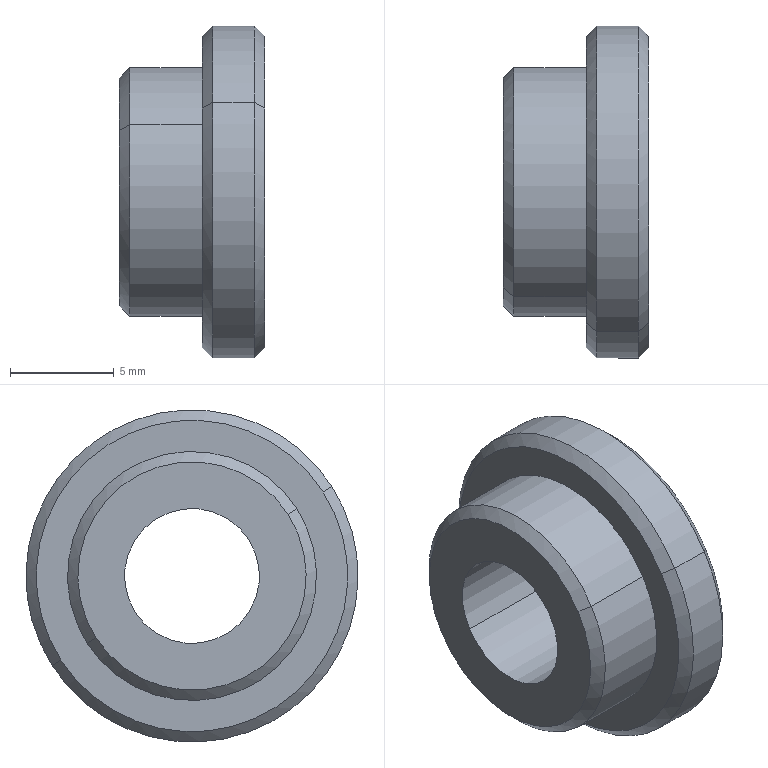Component | SolidWorks | RetainingRing-1 | 1 solid | 15 faces | box 7 x 16 x 16 mm | volume 806 mm3 | cone 6 | cylinder 6 | plane 3 | commonest cylinder face diameters 12 x2 16 x2 6.5 x2
build123d program:
from build123d import *


with BuildPart() as part:
    # Sketch1 → Revolve1 (revolve)
    with BuildSketch(Plane(origin=(0, 0, 0), x_dir=(0, 0, -1), z_dir=(1, 0, 0)), mode=Mode.PRIVATE) as revolve1_sk:
        Polygon((0, 3.25), (0, 7.5), (0.5, 8), (2.5, 8), (3, 7.5), (3, 6), (6.5, 6), (7, 5.5), (7, 3.25), align=None)
    revolve(revolve1_sk.sketch.rotate(Axis((0, 0, 0), (0, 0, -1)), 90), axis=Axis((0, 0, 0), (0, 0, -1)))


solid = part.part

# Placed as in the assembly
solid = solid.moved(Location((120.296, 56.837, 344.838), (0, 90, 0)))
STEP:
#1=COLOUR_RGB('',0.7922,0.8196,0.9333);
#2=FILL_AREA_STYLE_COLOUR('',#1);
#3=FILL_AREA_STYLE('',(#2));
#4=SURFACE_STYLE_FILL_AREA(#3);
#5=SURFACE_SIDE_STYLE('',(#4));
#6=SURFACE_STYLE_USAGE(.BOTH.,#5);
#7=PRESENTATION_STYLE_ASSIGNMENT((#6));
#8=CARTESIAN_POINT('',(4.46,2.055,13.693));
#9=VERTEX_POINT('',#8);
#10=CARTESIAN_POINT('',(4.46,2.42,13.459));
#11=VERTEX_POINT('',#10);
#12=CARTESIAN_POINT('',(4.46,2.238,13.576));
#13=DIRECTION('',(1.,0.,-0.));
#14=DIRECTION('',(0.,-0.8419,0.5397));
#15=AXIS2_PLACEMENT_3D('',#12,#13,#14);
#16=CIRCLE('',#15,0.2165);
#17=EDGE_CURVE('',#9,#11,#16,.T.);
#18=ORIENTED_EDGE('',*,*,#17,.T.);
#19=CARTESIAN_POINT('',(4.48,2.437,13.449));
#20=VERTEX_POINT('',#19);
#21=CARTESIAN_POINT('',(4.46,2.42,13.459));
#22=DIRECTION('',(0.7071,0.5953,-0.3816));
#23=VECTOR('',#22,39.37);
#24=LINE('',#21,#23);
#25=EDGE_CURVE('',#11,#20,#24,.T.);
#26=ORIENTED_EDGE('',*,*,#25,.T.);
#27=CARTESIAN_POINT('',(4.48,2.039,13.704));
#28=VERTEX_POINT('',#27);
#29=CARTESIAN_POINT('',(4.48,2.238,13.576));
#30=DIRECTION('',(1.,0.,-0.));
#31=DIRECTION('',(0.,-0.8419,0.5397));
#32=AXIS2_PLACEMENT_3D('',#29,#30,#31);
#33=CIRCLE('',#32,0.2362);
#34=EDGE_CURVE('',#28,#20,#33,.T.);
#35=ORIENTED_EDGE('',*,*,#34,.F.);
#36=CARTESIAN_POINT('',(4.46,2.055,13.693));
#37=DIRECTION('',(0.7071,-0.5953,0.3816));
#38=VECTOR('',#37,39.37);
#39=LINE('',#36,#38);
#40=EDGE_CURVE('',#9,#28,#39,.T.);
#41=ORIENTED_EDGE('',*,*,#40,.F.);
#42=EDGE_LOOP('',(#18,#26,#35,#41));
#43=FACE_OUTER_BOUND('',#42,.T.);
#44=CARTESIAN_POINT('',(4.46,2.238,13.576));
#45=DIRECTION('',(1.,0.,-0.));
#46=DIRECTION('',(0.,-0.8419,0.5397));
#47=AXIS2_PLACEMENT_3D('',#44,#45,#46);
#48=CONICAL_SURFACE('',#47,0.2165,0.7854);
#49=ADVANCED_FACE('',(#43),#48,.T.);
#50=ORIENTED_EDGE('',*,*,#34,.T.);
#51=CARTESIAN_POINT('',(4.618,2.437,13.449));
#52=VERTEX_POINT('',#51);
#53=CARTESIAN_POINT('',(4.736,2.437,13.449));
#54=DIRECTION('',(1.,0.,-0.));
#55=VECTOR('',#54,39.37);
#56=LINE('',#53,#55);
#57=EDGE_CURVE('',#20,#52,#56,.T.);
#58=ORIENTED_EDGE('',*,*,#57,.T.);
#59=CARTESIAN_POINT('',(4.618,2.039,13.704));
#60=VERTEX_POINT('',#59);
#61=CARTESIAN_POINT('',(4.618,2.238,13.576));
#62=DIRECTION('',(1.,0.,-0.));
#63=DIRECTION('',(0.,-0.8419,0.5397));
#64=AXIS2_PLACEMENT_3D('',#61,#62,#63);
#65=CIRCLE('',#64,0.2362);
#66=EDGE_CURVE('',#60,#52,#65,.T.);
#67=ORIENTED_EDGE('',*,*,#66,.F.);
#68=CARTESIAN_POINT('',(4.736,2.039,13.704));
#69=DIRECTION('',(1.,0.,-0.));
#70=VECTOR('',#69,39.37);
#71=LINE('',#68,#70);
#72=EDGE_CURVE('',#28,#60,#71,.T.);
#73=ORIENTED_EDGE('',*,*,#72,.F.);
#74=EDGE_LOOP('',(#50,#58,#67,#73));
#75=FACE_OUTER_BOUND('',#74,.T.);
#76=CARTESIAN_POINT('',(4.736,2.238,13.576));
#77=DIRECTION('',(1.,0.,-0.));
#78=DIRECTION('',(0.,-0.8419,0.5397));
#79=AXIS2_PLACEMENT_3D('',#76,#77,#78);
#80=CYLINDRICAL_SURFACE('',#79,0.2362);
#81=ADVANCED_FACE('',(#75),#80,.T.);
#82=CARTESIAN_POINT('',(4.618,1.989,13.736));
#83=VERTEX_POINT('',#82);
#84=CARTESIAN_POINT('',(4.618,2.486,13.417));
#85=VERTEX_POINT('',#84);
#86=CARTESIAN_POINT('',(4.618,2.238,13.576));
#87=DIRECTION('',(1.,0.,-0.));
#88=DIRECTION('',(0.,-0.8419,0.5397));
#89=AXIS2_PLACEMENT_3D('',#86,#87,#88);
#90=CIRCLE('',#89,0.2953);
#91=EDGE_CURVE('',#83,#85,#90,.T.);
#92=ORIENTED_EDGE('',*,*,#91,.T.);
#93=CARTESIAN_POINT('',(4.638,2.503,13.406));
#94=VERTEX_POINT('',#93);
#95=CARTESIAN_POINT('',(4.618,2.486,13.417));
#96=DIRECTION('',(0.7071,0.5953,-0.3816));
#97=VECTOR('',#96,39.37);
#98=LINE('',#95,#97);
#99=EDGE_CURVE('',#85,#94,#98,.T.);
#100=ORIENTED_EDGE('',*,*,#99,.T.);
#101=CARTESIAN_POINT('',(4.638,1.973,13.746));
#102=VERTEX_POINT('',#101);
#103=CARTESIAN_POINT('',(4.638,2.238,13.576));
#104=DIRECTION('',(1.,0.,-0.));
#105=DIRECTION('',(0.,-0.8419,0.5397));
#106=AXIS2_PLACEMENT_3D('',#103,#104,#105);
#107=CIRCLE('',#106,0.315);
#108=EDGE_CURVE('',#102,#94,#107,.T.);
#109=ORIENTED_EDGE('',*,*,#108,.F.);
#110=CARTESIAN_POINT('',(4.618,1.989,13.736));
#111=DIRECTION('',(0.7071,-0.5953,0.3816));
#112=VECTOR('',#111,39.37);
#113=LINE('',#110,#112);
#114=EDGE_CURVE('',#83,#102,#113,.T.);
#115=ORIENTED_EDGE('',*,*,#114,.F.);
#116=EDGE_LOOP('',(#92,#100,#109,#115));
#117=FACE_OUTER_BOUND('',#116,.T.);
#118=CARTESIAN_POINT('',(4.618,2.238,13.576));
#119=DIRECTION('',(1.,0.,-0.));
#120=DIRECTION('',(0.,-0.8419,0.5397));
#121=AXIS2_PLACEMENT_3D('',#118,#119,#120);
#122=CONICAL_SURFACE('',#121,0.2953,0.7854);
#123=ADVANCED_FACE('',(#117),#122,.T.);
#124=ORIENTED_EDGE('',*,*,#108,.T.);
#125=CARTESIAN_POINT('',(4.716,2.503,13.406));
#126=VERTEX_POINT('',#125);
#127=CARTESIAN_POINT('',(4.736,2.503,13.406));
#128=DIRECTION('',(1.,0.,-0.));
#129=VECTOR('',#128,39.37);
#130=LINE('',#127,#129);
#131=EDGE_CURVE('',#94,#126,#130,.T.);
#132=ORIENTED_EDGE('',*,*,#131,.T.);
#133=CARTESIAN_POINT('',(4.716,1.973,13.746));
#134=VERTEX_POINT('',#133);
#135=CARTESIAN_POINT('',(4.716,2.238,13.576));
#136=DIRECTION('',(1.,0.,-0.));
#137=DIRECTION('',(0.,-0.8419,0.5397));
#138=AXIS2_PLACEMENT_3D('',#135,#136,#137);
#139=CIRCLE('',#138,0.315);
#140=EDGE_CURVE('',#134,#126,#139,.T.);
#141=ORIENTED_EDGE('',*,*,#140,.F.);
#142=CARTESIAN_POINT('',(4.736,1.973,13.746));
#143=DIRECTION('',(1.,0.,-0.));
#144=VECTOR('',#143,39.37);
#145=LINE('',#142,#144);
#146=EDGE_CURVE('',#102,#134,#145,.T.);
#147=ORIENTED_EDGE('',*,*,#146,.F.);
#148=EDGE_LOOP('',(#124,#132,#141,#147));
#149=FACE_OUTER_BOUND('',#148,.T.);
#150=CARTESIAN_POINT('',(4.736,2.238,13.576));
#151=DIRECTION('',(1.,0.,-0.));
#152=DIRECTION('',(0.,-0.8419,0.5397));
#153=AXIS2_PLACEMENT_3D('',#150,#151,#152);
#154=CYLINDRICAL_SURFACE('',#153,0.315);
#155=ADVANCED_FACE('',(#149),#154,.T.);
#156=CARTESIAN_POINT('',(4.736,1.989,13.736));
#157=VERTEX_POINT('',#156);
#158=CARTESIAN_POINT('',(4.736,2.486,13.417));
#159=VERTEX_POINT('',#158);
#160=CARTESIAN_POINT('',(4.736,2.238,13.576));
#161=DIRECTION('',(1.,0.,-0.));
#162=DIRECTION('',(0.,-0.8419,0.5397));
#163=AXIS2_PLACEMENT_3D('',#160,#161,#162);
#164=CIRCLE('',#163,0.2953);
#165=EDGE_CURVE('',#157,#159,#164,.T.);
#166=ORIENTED_EDGE('',*,*,#165,.F.);
#167=CARTESIAN_POINT('',(4.716,1.973,13.746));
#168=DIRECTION('',(-0.7071,-0.5953,0.3816));
#169=VECTOR('',#168,39.37);
#170=LINE('',#167,#169);
#171=EDGE_CURVE('',#157,#134,#170,.T.);
#172=ORIENTED_EDGE('',*,*,#171,.T.);
#173=ORIENTED_EDGE('',*,*,#140,.T.);
#174=CARTESIAN_POINT('',(4.716,2.503,13.406));
#175=DIRECTION('',(-0.7071,0.5953,-0.3816));
#176=VECTOR('',#175,39.37);
#177=LINE('',#174,#176);
#178=EDGE_CURVE('',#159,#126,#177,.T.);
#179=ORIENTED_EDGE('',*,*,#178,.F.);
#180=EDGE_LOOP('',(#166,#172,#173,#179));
#181=FACE_OUTER_BOUND('',#180,.T.);
#182=CARTESIAN_POINT('',(4.716,2.238,13.576));
#183=DIRECTION('',(-1.,-0.,0.));
#184=DIRECTION('',(-0.,0.8419,-0.5397));
#185=AXIS2_PLACEMENT_3D('',#182,#183,#184);
#186=CONICAL_SURFACE('',#185,0.315,0.7854);
#187=ADVANCED_FACE('',(#181),#186,.T.);
#188=CARTESIAN_POINT('',(4.46,2.345,13.507));
#189=VERTEX_POINT('',#188);
#190=CARTESIAN_POINT('',(4.46,2.13,13.645));
#191=VERTEX_POINT('',#190);
#192=CARTESIAN_POINT('',(4.46,2.238,13.576));
#193=DIRECTION('',(1.,0.,-0.));
#194=DIRECTION('',(0.,-0.8419,0.5397));
#195=AXIS2_PLACEMENT_3D('',#192,#193,#194);
#196=CIRCLE('',#195,0.128);
#197=EDGE_CURVE('',#189,#191,#196,.T.);
#198=ORIENTED_EDGE('',*,*,#197,.F.);
#199=CARTESIAN_POINT('',(4.736,2.345,13.507));
#200=VERTEX_POINT('',#199);
#201=CARTESIAN_POINT('',(4.736,2.345,13.507));
#202=DIRECTION('',(1.,0.,-0.));
#203=VECTOR('',#202,39.37);
#204=LINE('',#201,#203);
#205=EDGE_CURVE('',#189,#200,#204,.T.);
#206=ORIENTED_EDGE('',*,*,#205,.T.);
#207=CARTESIAN_POINT('',(4.736,2.13,13.645));
#208=VERTEX_POINT('',#207);
#209=CARTESIAN_POINT('',(4.736,2.238,13.576));
#210=DIRECTION('',(1.,0.,-0.));
#211=DIRECTION('',(0.,-0.8419,0.5397));
#212=AXIS2_PLACEMENT_3D('',#209,#210,#211);
#213=CIRCLE('',#212,0.128);
#214=EDGE_CURVE('',#200,#208,#213,.T.);
#215=ORIENTED_EDGE('',*,*,#214,.T.);
#216=CARTESIAN_POINT('',(4.736,2.13,13.645));
#217=DIRECTION('',(1.,0.,-0.));
#218=VECTOR('',#217,39.37);
#219=LINE('',#216,#218);
#220=EDGE_CURVE('',#191,#208,#219,.T.);
#221=ORIENTED_EDGE('',*,*,#220,.F.);
#222=EDGE_LOOP('',(#198,#206,#215,#221));
#223=FACE_OUTER_BOUND('',#222,.T.);
#224=CARTESIAN_POINT('',(4.736,2.238,13.576));
#225=DIRECTION('',(1.,0.,-0.));
#226=DIRECTION('',(0.,-0.8419,0.5397));
#227=AXIS2_PLACEMENT_3D('',#224,#225,#226);
#228=CYLINDRICAL_SURFACE('',#227,0.128);
#229=ADVANCED_FACE('',(#223),#228,.F.);
#230=ORIENTED_EDGE('',*,*,#205,.F.);
#231=CARTESIAN_POINT('',(4.46,2.238,13.576));
#232=DIRECTION('',(1.,0.,-0.));
#233=DIRECTION('',(0.,-0.8419,0.5397));
#234=AXIS2_PLACEMENT_3D('',#231,#232,#233);
#235=CIRCLE('',#234,0.128);
#236=EDGE_CURVE('',#191,#189,#235,.T.);
#237=ORIENTED_EDGE('',*,*,#236,.F.);
#238=ORIENTED_EDGE('',*,*,#220,.T.);
#239=CARTESIAN_POINT('',(4.736,2.238,13.576));
#240=DIRECTION('',(1.,0.,-0.));
#241=DIRECTION('',(0.,-0.8419,0.5397));
#242=AXIS2_PLACEMENT_3D('',#239,#240,#241);
#243=CIRCLE('',#242,0.128);
#244=EDGE_CURVE('',#208,#200,#243,.T.);
#245=ORIENTED_EDGE('',*,*,#244,.T.);
#246=EDGE_LOOP('',(#230,#237,#238,#245));
#247=FACE_OUTER_BOUND('',#246,.T.);
#248=CARTESIAN_POINT('',(4.736,2.238,13.576));
#249=DIRECTION('',(1.,0.,-0.));
#250=DIRECTION('',(0.,-0.8419,0.5397));
#251=AXIS2_PLACEMENT_3D('',#248,#249,#250);
#252=CYLINDRICAL_SURFACE('',#251,0.128);
#253=ADVANCED_FACE('',(#247),#252,.F.);
#254=ORIENTED_EDGE('',*,*,#244,.F.);
#255=ORIENTED_EDGE('',*,*,#214,.F.);
#256=EDGE_LOOP('',(#254,#255));
#257=FACE_BOUND('',#256,.T.);
#258=CARTESIAN_POINT('',(4.736,2.238,13.576));
#259=DIRECTION('',(1.,0.,-0.));
#260=DIRECTION('',(0.,-0.8419,0.5397));
#261=AXIS2_PLACEMENT_3D('',#258,#259,#260);
#262=CIRCLE('',#261,0.2953);
#263=EDGE_CURVE('',#159,#157,#262,.T.);
#264=ORIENTED_EDGE('',*,*,#263,.T.);
#265=ORIENTED_EDGE('',*,*,#165,.T.);
#266=EDGE_LOOP('',(#264,#265));
#267=FACE_OUTER_BOUND('',#266,.T.);
#268=CARTESIAN_POINT('',(4.736,2.169,13.469));
#269=DIRECTION('',(-1.,-0.,0.));
#270=DIRECTION('',(-0.,0.8419,-0.5397));
#271=AXIS2_PLACEMENT_3D('',#268,#269,#270);
#272=PLANE('',#271);
#273=ADVANCED_FACE('',(#257,#267),#272,.F.);
#274=ORIENTED_EDGE('',*,*,#171,.F.);
#275=ORIENTED_EDGE('',*,*,#263,.F.);
#276=ORIENTED_EDGE('',*,*,#178,.T.);
#277=CARTESIAN_POINT('',(4.716,2.238,13.576));
#278=DIRECTION('',(1.,0.,-0.));
#279=DIRECTION('',(0.,-0.8419,0.5397));
#280=AXIS2_PLACEMENT_3D('',#277,#278,#279);
#281=CIRCLE('',#280,0.315);
#282=EDGE_CURVE('',#126,#134,#281,.T.);
#283=ORIENTED_EDGE('',*,*,#282,.T.);
#284=EDGE_LOOP('',(#274,#275,#276,#283));
#285=FACE_OUTER_BOUND('',#284,.T.);
#286=CARTESIAN_POINT('',(4.716,2.238,13.576));
#287=DIRECTION('',(-1.,-0.,0.));
#288=DIRECTION('',(-0.,0.8419,-0.5397));
#289=AXIS2_PLACEMENT_3D('',#286,#287,#288);
#290=CONICAL_SURFACE('',#289,0.315,0.7854);
#291=ADVANCED_FACE('',(#285),#290,.T.);
#292=ORIENTED_EDGE('',*,*,#131,.F.);
#293=CARTESIAN_POINT('',(4.638,2.238,13.576));
#294=DIRECTION('',(1.,0.,-0.));
#295=DIRECTION('',(0.,-0.8419,0.5397));
#296=AXIS2_PLACEMENT_3D('',#293,#294,#295);
#297=CIRCLE('',#296,0.315);
#298=EDGE_CURVE('',#94,#102,#297,.T.);
#299=ORIENTED_EDGE('',*,*,#298,.T.);
#300=ORIENTED_EDGE('',*,*,#146,.T.);
#301=ORIENTED_EDGE('',*,*,#282,.F.);
#302=EDGE_LOOP('',(#292,#299,#300,#301));
#303=FACE_OUTER_BOUND('',#302,.T.);
#304=CARTESIAN_POINT('',(4.736,2.238,13.576));
#305=DIRECTION('',(1.,0.,-0.));
#306=DIRECTION('',(0.,-0.8419,0.5397));
#307=AXIS2_PLACEMENT_3D('',#304,#305,#306);
#308=CYLINDRICAL_SURFACE('',#307,0.315);
#309=ADVANCED_FACE('',(#303),#308,.T.);
#310=ORIENTED_EDGE('',*,*,#99,.F.);
#311=CARTESIAN_POINT('',(4.618,2.238,13.576));
#312=DIRECTION('',(1.,0.,-0.));
#313=DIRECTION('',(0.,-0.8419,0.5397));
#314=AXIS2_PLACEMENT_3D('',#311,#312,#313);
#315=CIRCLE('',#314,0.2953);
#316=EDGE_CURVE('',#85,#83,#315,.T.);
#317=ORIENTED_EDGE('',*,*,#316,.T.);
#318=ORIENTED_EDGE('',*,*,#114,.T.);
#319=ORIENTED_EDGE('',*,*,#298,.F.);
#320=EDGE_LOOP('',(#310,#317,#318,#319));
#321=FACE_OUTER_BOUND('',#320,.T.);
#322=CARTESIAN_POINT('',(4.618,2.238,13.576));
#323=DIRECTION('',(1.,0.,-0.));
#324=DIRECTION('',(0.,-0.8419,0.5397));
#325=AXIS2_PLACEMENT_3D('',#322,#323,#324);
#326=CONICAL_SURFACE('',#325,0.2953,0.7854);
#327=ADVANCED_FACE('',(#321),#326,.T.);
#328=ORIENTED_EDGE('',*,*,#91,.F.);
#329=ORIENTED_EDGE('',*,*,#316,.F.);
#330=EDGE_LOOP('',(#328,#329));
#331=FACE_OUTER_BOUND('',#330,.T.);
#332=ORIENTED_EDGE('',*,*,#66,.T.);
#333=CARTESIAN_POINT('',(4.618,2.238,13.576));
#334=DIRECTION('',(1.,0.,-0.));
#335=DIRECTION('',(0.,-0.8419,0.5397));
#336=AXIS2_PLACEMENT_3D('',#333,#334,#335);
#337=CIRCLE('',#336,0.2362);
#338=EDGE_CURVE('',#52,#60,#337,.T.);
#339=ORIENTED_EDGE('',*,*,#338,.T.);
#340=EDGE_LOOP('',(#332,#339));
#341=FACE_BOUND('',#340,.T.);
#342=CARTESIAN_POINT('',(4.618,2.078,13.328));
#343=DIRECTION('',(1.,0.,-0.));
#344=DIRECTION('',(0.,-0.8419,0.5397));
#345=AXIS2_PLACEMENT_3D('',#342,#343,#344);
#346=PLANE('',#345);
#347=ADVANCED_FACE('',(#331,#341),#346,.F.);
#348=ORIENTED_EDGE('',*,*,#57,.F.);
#349=CARTESIAN_POINT('',(4.48,2.238,13.576));
#350=DIRECTION('',(1.,0.,-0.));
#351=DIRECTION('',(0.,-0.8419,0.5397));
#352=AXIS2_PLACEMENT_3D('',#349,#350,#351);
#353=CIRCLE('',#352,0.2362);
#354=EDGE_CURVE('',#20,#28,#353,.T.);
#355=ORIENTED_EDGE('',*,*,#354,.T.);
#356=ORIENTED_EDGE('',*,*,#72,.T.);
#357=ORIENTED_EDGE('',*,*,#338,.F.);
#358=EDGE_LOOP('',(#348,#355,#356,#357));
#359=FACE_OUTER_BOUND('',#358,.T.);
#360=CARTESIAN_POINT('',(4.736,2.238,13.576));
#361=DIRECTION('',(1.,0.,-0.));
#362=DIRECTION('',(0.,-0.8419,0.5397));
#363=AXIS2_PLACEMENT_3D('',#360,#361,#362);
#364=CYLINDRICAL_SURFACE('',#363,0.2362);
#365=ADVANCED_FACE('',(#359),#364,.T.);
#366=ORIENTED_EDGE('',*,*,#25,.F.);
#367=CARTESIAN_POINT('',(4.46,2.238,13.576));
#368=DIRECTION('',(1.,0.,-0.));
#369=DIRECTION('',(0.,-0.8419,0.5397));
#370=AXIS2_PLACEMENT_3D('',#367,#368,#369);
#371=CIRCLE('',#370,0.2165);
#372=EDGE_CURVE('',#11,#9,#371,.T.);
#373=ORIENTED_EDGE('',*,*,#372,.T.);
#374=ORIENTED_EDGE('',*,*,#40,.T.);
#375=ORIENTED_EDGE('',*,*,#354,.F.);
#376=EDGE_LOOP('',(#366,#373,#374,#375));
#377=FACE_OUTER_BOUND('',#376,.T.);
#378=CARTESIAN_POINT('',(4.46,2.238,13.576));
#379=DIRECTION('',(1.,0.,-0.));
#380=DIRECTION('',(0.,-0.8419,0.5397));
#381=AXIS2_PLACEMENT_3D('',#378,#379,#380);
#382=CONICAL_SURFACE('',#381,0.2165,0.7854);
#383=ADVANCED_FACE('',(#377),#382,.T.);
#384=ORIENTED_EDGE('',*,*,#17,.F.);
#385=ORIENTED_EDGE('',*,*,#372,.F.);
#386=EDGE_LOOP('',(#384,#385));
#387=FACE_OUTER_BOUND('',#386,.T.);
#388=ORIENTED_EDGE('',*,*,#236,.T.);
#389=ORIENTED_EDGE('',*,*,#197,.T.);
#390=EDGE_LOOP('',(#388,#389));
#391=FACE_BOUND('',#390,.T.);
#392=CARTESIAN_POINT('',(4.46,2.121,13.394));
#393=DIRECTION('',(1.,0.,-0.));
#394=DIRECTION('',(0.,-0.8419,0.5397));
#395=AXIS2_PLACEMENT_3D('',#392,#393,#394);
#396=PLANE('',#395);
#397=ADVANCED_FACE('',(#387,#391),#396,.F.);
#398=CLOSED_SHELL('',(#49,#81,#123,#155,#187,#229,#253,#273,#291,#309,#327,#347,#365,#383,#397));
#399=MANIFOLD_SOLID_BREP('',#398);
#400=STYLED_ITEM('',(#7),#399);
#401=(LENGTH_UNIT()NAMED_UNIT(*)SI_UNIT($,.METRE.));
#402=LENGTH_MEASURE_WITH_UNIT(LENGTH_MEASURE(0.0254),#401);
#403=DIMENSIONAL_EXPONENTS(1.,0.,0.,0.,0.,0.,0.);
#404=(CONVERSION_BASED_UNIT('',#402)LENGTH_UNIT()NAMED_UNIT(#403));
#405=UNCERTAINTY_MEASURE_WITH_UNIT(LENGTH_MEASURE(0.00001),#404,'','');
#406=(NAMED_UNIT(*)PLANE_ANGLE_UNIT()SI_UNIT($,.RADIAN.));
#407=(NAMED_UNIT(*)SI_UNIT($,.STERADIAN.)SOLID_ANGLE_UNIT());
#408=(GEOMETRIC_REPRESENTATION_CONTEXT(3)GLOBAL_UNCERTAINTY_ASSIGNED_CONTEXT((#405))GLOBAL_UNIT_ASSIGNED_CONTEXT((#404,#406,#407))REPRESENTATION_CONTEXT('',''));
#409=MECHANICAL_DESIGN_GEOMETRIC_PRESENTATION_REPRESENTATION('',(#400),#408);
#410=CARTESIAN_POINT('',(0.,0.,0.));
#411=DIRECTION('',(0.,0.,1.));
#412=DIRECTION('',(1.,0.,0.));
#413=AXIS2_PLACEMENT_3D('',#410,#411,#412);
#414=(LENGTH_UNIT()NAMED_UNIT(*)SI_UNIT($,.METRE.));
#415=LENGTH_MEASURE_WITH_UNIT(LENGTH_MEASURE(0.0254),#414);
#416=DIMENSIONAL_EXPONENTS(1.,0.,0.,0.,0.,0.,0.);
#417=(CONVERSION_BASED_UNIT('',#415)LENGTH_UNIT()NAMED_UNIT(#416));
#418=UNCERTAINTY_MEASURE_WITH_UNIT(LENGTH_MEASURE(0.00001),#417,'','');
#419=(NAMED_UNIT(*)PLANE_ANGLE_UNIT()SI_UNIT($,.RADIAN.));
#420=(NAMED_UNIT(*)SI_UNIT($,.STERADIAN.)SOLID_ANGLE_UNIT());
#421=(GEOMETRIC_REPRESENTATION_CONTEXT(3)GLOBAL_UNCERTAINTY_ASSIGNED_CONTEXT((#418))GLOBAL_UNIT_ASSIGNED_CONTEXT((#417,#419,#420))REPRESENTATION_CONTEXT('',''));
#422=ADVANCED_BREP_SHAPE_REPRESENTATION('',(#399,#413),#421);
#423=PRESENTATION_LAYER_ASSIGNMENT('','',(#400));